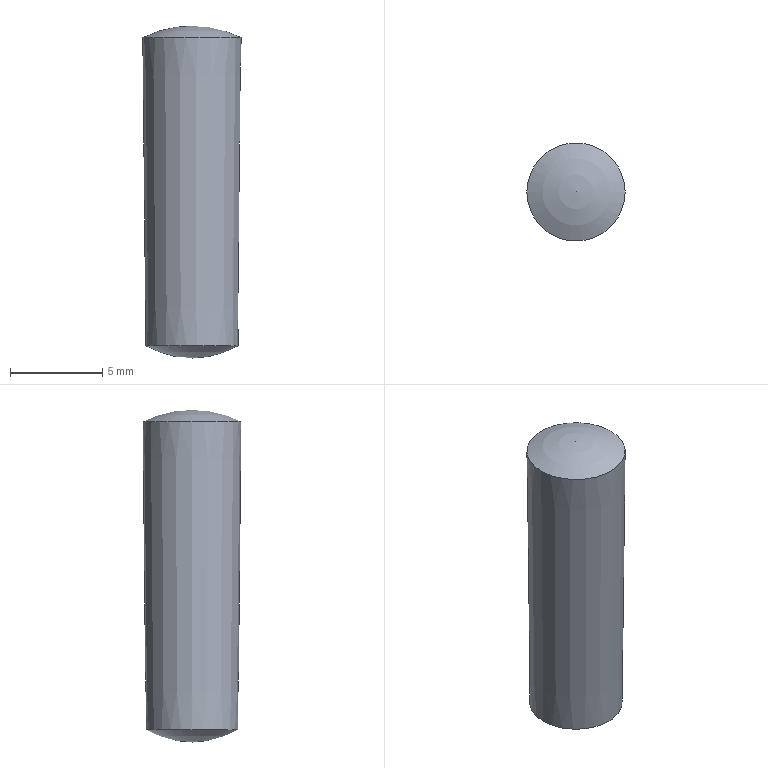Component | NX | GB-T117_A-2000_5X18 | 1 solid | 3 faces | box 5.33 x 5.33 x 18 mm | volume 364 mm3 | sphere 2 | cone 1
STEP:
#1=CARTESIAN_POINT('',(0.,0.,0.));
#2=DIRECTION('',(0.,0.,1.));
#3=DIRECTION('',(1.,0.,0.));
#4=AXIS2_PLACEMENT_3D('',#1,#2,#3);
#5=CARTESIAN_POINT('',(31.561,-84.527,-162.349));
#6=VERTEX_POINT('',#5);
#7=CARTESIAN_POINT('',(34.228,-84.527,-162.349));
#8=DIRECTION('',(0.,0.,-1.));
#9=DIRECTION('',(-1.,0.,0.));
#10=AXIS2_PLACEMENT_3D('',#7,#8,#9);
#11=CIRCLE('',#10,2.667);
#12=CARTESIAN_POINT('',(34.228,-84.527,-167.679));
#13=DIRECTION('',(0.,0.,-1.));
#14=DIRECTION('',(-1.,0.,0.));
#15=AXIS2_PLACEMENT_3D('',#12,#13,#14);
#16=SPHERICAL_SURFACE('',#15,5.96);
#17=CARTESIAN_POINT('',(0.,-1.107));
#18=CARTESIAN_POINT('',(0.0952,-1.107));
#19=CARTESIAN_POINT('',(0.2856,-1.107));
#20=CARTESIAN_POINT('',(0.5712,-1.107));
#21=CARTESIAN_POINT('',(0.8568,-1.107));
#22=CARTESIAN_POINT('',(1.142,-1.107));
#23=CARTESIAN_POINT('',(1.428,-1.107));
#24=CARTESIAN_POINT('',(1.714,-1.107));
#25=CARTESIAN_POINT('',(1.999,-1.107));
#26=CARTESIAN_POINT('',(2.285,-1.107));
#27=CARTESIAN_POINT('',(2.57,-1.107));
#28=CARTESIAN_POINT('',(2.856,-1.107));
#29=CARTESIAN_POINT('',(3.142,-1.107));
#30=CARTESIAN_POINT('',(3.427,-1.107));
#31=CARTESIAN_POINT('',(3.713,-1.107));
#32=CARTESIAN_POINT('',(3.998,-1.107));
#33=CARTESIAN_POINT('',(4.284,-1.107));
#34=CARTESIAN_POINT('',(4.57,-1.107));
#35=CARTESIAN_POINT('',(4.855,-1.107));
#36=CARTESIAN_POINT('',(5.141,-1.107));
#37=CARTESIAN_POINT('',(5.426,-1.107));
#38=CARTESIAN_POINT('',(5.712,-1.107));
#39=CARTESIAN_POINT('',(5.998,-1.107));
#40=CARTESIAN_POINT('',(6.188,-1.107));
#41=CARTESIAN_POINT('',(6.283,-1.107));
#42=B_SPLINE_CURVE_WITH_KNOTS('',3,(#17,#18,#19,#20,#21,#22,#23,#24,#25,#26,#27,#28,#29,#30,#31,#32,#33,#34,#35,#36,#37,#38,#39,#40,#41),.UNSPECIFIED.,.F.,.F.,(4,1,1,1,1,1,1,1,1,1,1,1,1,1,1,1,1,1,1,1,1,1,4),(0.,0.2856,0.5712,0.8568,1.142,1.428,1.714,1.999,2.285,2.57,2.856,3.142,3.427,3.713,3.998,4.284,4.57,4.855,5.141,5.426,5.712,5.998,6.283),.QUASI_UNIFORM_KNOTS.);
#43=(GEOMETRIC_REPRESENTATION_CONTEXT(2)PARAMETRIC_REPRESENTATION_CONTEXT()REPRESENTATION_CONTEXT('',''));
#44=DEFINITIONAL_REPRESENTATION('',(#42),#43);
#45=PCURVE('',#16,#44);
#46=CARTESIAN_POINT('',(34.228,-84.527,-162.349));
#47=DIRECTION('',(0.,0.,1.));
#48=DIRECTION('',(1.,0.,0.));
#49=AXIS2_PLACEMENT_3D('',#46,#47,#48);
#50=CONICAL_SURFACE('',#49,2.667,0.01);
#51=CARTESIAN_POINT('',(9.425,0.));
#52=DIRECTION('',(-1.,0.));
#53=VECTOR('',#52,1.);
#54=LINE('',#51,#53);
#55=(GEOMETRIC_REPRESENTATION_CONTEXT(2)PARAMETRIC_REPRESENTATION_CONTEXT()REPRESENTATION_CONTEXT('',''));
#56=DEFINITIONAL_REPRESENTATION('',(#54),#55);
#57=PCURVE('',#50,#56);
#58=SURFACE_CURVE('',#11,(#45,#57),.PCURVE_S1.);
#59=EDGE_CURVE('',#6,#6,#58,.T.);
#60=ORIENTED_EDGE('',*,*,#59,.F.);
#61=CARTESIAN_POINT('',(34.228,-84.527,-161.719));
#62=VERTEX_POINT('',#61);
#63=CARTESIAN_POINT('',(34.228,-84.527,-161.719));
#64=CARTESIAN_POINT('',(33.537,-84.527,-161.719));
#65=CARTESIAN_POINT('',(32.846,-84.527,-161.826));
#66=CARTESIAN_POINT('',(32.179,-84.527,-162.04));
#67=CARTESIAN_POINT('',(31.561,-84.527,-162.349));
#68=B_SPLINE_CURVE_WITH_KNOTS('',4,(#63,#64,#65,#66,#67),.UNSPECIFIED.,.F.,.F.,(5,5),(-1.571,-1.107),.PIECEWISE_BEZIER_KNOTS.);
#69=CARTESIAN_POINT('',(0.,0.));
#70=DIRECTION('',(0.,1.));
#71=VECTOR('',#70,1.);
#72=LINE('',#69,#71);
#73=(GEOMETRIC_REPRESENTATION_CONTEXT(2)PARAMETRIC_REPRESENTATION_CONTEXT()REPRESENTATION_CONTEXT('',''));
#74=DEFINITIONAL_REPRESENTATION('',(#72),#73);
#75=PCURVE('',#16,#74);
#76=CARTESIAN_POINT('',(6.283,0.));
#77=DIRECTION('',(0.,1.));
#78=VECTOR('',#77,1.);
#79=LINE('',#76,#78);
#80=(GEOMETRIC_REPRESENTATION_CONTEXT(2)PARAMETRIC_REPRESENTATION_CONTEXT()REPRESENTATION_CONTEXT('',''));
#81=DEFINITIONAL_REPRESENTATION('',(#79),#80);
#82=PCURVE('',#16,#81);
#83=SEAM_CURVE('',#68,(#75,#82),.PCURVE_S1.);
#84=EDGE_CURVE('',#62,#6,#83,.T.);
#85=ORIENTED_EDGE('',*,*,#84,.F.);
#86=ORIENTED_EDGE('',*,*,#84,.T.);
#87=EDGE_LOOP('',(#60,#85,#86));
#88=FACE_BOUND('',#87,.T.);
#89=ADVANCED_FACE('',(#88),#16,.T.);
#90=CARTESIAN_POINT('',(31.728,-84.527,-179.049));
#91=VERTEX_POINT('',#90);
#92=CARTESIAN_POINT('',(36.728,-84.527,-179.049));
#93=VERTEX_POINT('',#92);
#94=CARTESIAN_POINT('',(34.228,-84.527,-179.049));
#95=DIRECTION('',(0.,0.,-1.));
#96=DIRECTION('',(-1.,0.,0.));
#97=AXIS2_PLACEMENT_3D('',#94,#95,#96);
#98=CIRCLE('',#97,2.5);
#99=CARTESIAN_POINT('',(9.425,-16.7));
#100=DIRECTION('',(-1.,0.));
#101=VECTOR('',#100,1.);
#102=LINE('',#99,#101);
#103=(GEOMETRIC_REPRESENTATION_CONTEXT(2)PARAMETRIC_REPRESENTATION_CONTEXT()REPRESENTATION_CONTEXT('',''));
#104=DEFINITIONAL_REPRESENTATION('',(#102),#103);
#105=PCURVE('',#50,#104);
#106=CARTESIAN_POINT('',(34.228,-84.527,-174.719));
#107=DIRECTION('',(0.,0.,-1.));
#108=DIRECTION('',(1.,0.,0.));
#109=AXIS2_PLACEMENT_3D('',#106,#107,#108);
#110=SPHERICAL_SURFACE('',#109,5.);
#111=CARTESIAN_POINT('',(3.142,1.047));
#112=CARTESIAN_POINT('',(3.237,1.047));
#113=CARTESIAN_POINT('',(3.427,1.047));
#114=CARTESIAN_POINT('',(3.713,1.047));
#115=CARTESIAN_POINT('',(3.998,1.047));
#116=CARTESIAN_POINT('',(4.284,1.047));
#117=CARTESIAN_POINT('',(4.57,1.047));
#118=CARTESIAN_POINT('',(4.855,1.047));
#119=CARTESIAN_POINT('',(5.141,1.047));
#120=CARTESIAN_POINT('',(5.426,1.047));
#121=CARTESIAN_POINT('',(5.712,1.047));
#122=CARTESIAN_POINT('',(5.998,1.047));
#123=CARTESIAN_POINT('',(6.283,1.047));
#124=CARTESIAN_POINT('',(6.569,1.047));
#125=CARTESIAN_POINT('',(6.854,1.047));
#126=CARTESIAN_POINT('',(7.14,1.047));
#127=CARTESIAN_POINT('',(7.426,1.047));
#128=CARTESIAN_POINT('',(7.711,1.047));
#129=CARTESIAN_POINT('',(7.997,1.047));
#130=CARTESIAN_POINT('',(8.282,1.047));
#131=CARTESIAN_POINT('',(8.568,1.047));
#132=CARTESIAN_POINT('',(8.854,1.047));
#133=CARTESIAN_POINT('',(9.139,1.047));
#134=CARTESIAN_POINT('',(9.33,1.047));
#135=CARTESIAN_POINT('',(9.425,1.047));
#136=B_SPLINE_CURVE_WITH_KNOTS('',3,(#111,#112,#113,#114,#115,#116,#117,#118,#119,#120,#121,#122,#123,#124,#125,#126,#127,#128,#129,#130,#131,#132,#133,#134,#135),.UNSPECIFIED.,.F.,.F.,(4,1,1,1,1,1,1,1,1,1,1,1,1,1,1,1,1,1,1,1,1,1,4),(0.,0.2856,0.5712,0.8568,1.142,1.428,1.714,1.999,2.285,2.57,2.856,3.142,3.427,3.713,3.998,4.284,4.57,4.855,5.141,5.426,5.712,5.998,6.283),.QUASI_UNIFORM_KNOTS.);
#137=(GEOMETRIC_REPRESENTATION_CONTEXT(2)PARAMETRIC_REPRESENTATION_CONTEXT()REPRESENTATION_CONTEXT('',''));
#138=DEFINITIONAL_REPRESENTATION('',(#136),#137);
#139=PCURVE('',#110,#138);
#140=SURFACE_CURVE('',#98,(#105,#139),.PCURVE_S1.);
#141=EDGE_CURVE('',#91,#93,#140,.T.);
#142=ORIENTED_EDGE('',*,*,#141,.F.);
#143=CARTESIAN_POINT('',(31.728,-84.527,-179.049));
#144=CARTESIAN_POINT('',(31.561,-84.527,-162.349));
#145=B_SPLINE_CURVE_WITH_KNOTS('',1,(#143,#144),.UNSPECIFIED.,.F.,.F.,(2,2),(-16.701,0.),.PIECEWISE_BEZIER_KNOTS.);
#146=CARTESIAN_POINT('',(9.425,0.));
#147=DIRECTION('',(0.,1.));
#148=VECTOR('',#147,1.);
#149=LINE('',#146,#148);
#150=(GEOMETRIC_REPRESENTATION_CONTEXT(2)PARAMETRIC_REPRESENTATION_CONTEXT()REPRESENTATION_CONTEXT('',''));
#151=DEFINITIONAL_REPRESENTATION('',(#149),#150);
#152=PCURVE('',#50,#151);
#153=CARTESIAN_POINT('',(3.142,0.));
#154=DIRECTION('',(0.,1.));
#155=VECTOR('',#154,1.);
#156=LINE('',#153,#155);
#157=(GEOMETRIC_REPRESENTATION_CONTEXT(2)PARAMETRIC_REPRESENTATION_CONTEXT()REPRESENTATION_CONTEXT('',''));
#158=DEFINITIONAL_REPRESENTATION('',(#156),#157);
#159=PCURVE('',#50,#158);
#160=SEAM_CURVE('',#145,(#152,#159),.PCURVE_S1.);
#161=EDGE_CURVE('',#91,#6,#160,.T.);
#162=ORIENTED_EDGE('',*,*,#161,.T.);
#163=ORIENTED_EDGE('',*,*,#59,.T.);
#164=ORIENTED_EDGE('',*,*,#161,.F.);
#165=CARTESIAN_POINT('',(34.228,-84.527,-179.049));
#166=DIRECTION('',(0.,0.,-1.));
#167=DIRECTION('',(-1.,0.,0.));
#168=AXIS2_PLACEMENT_3D('',#165,#166,#167);
#169=CIRCLE('',#168,2.5);
#170=CARTESIAN_POINT('',(9.425,-16.7));
#171=DIRECTION('',(-1.,0.));
#172=VECTOR('',#171,1.);
#173=LINE('',#170,#172);
#174=(GEOMETRIC_REPRESENTATION_CONTEXT(2)PARAMETRIC_REPRESENTATION_CONTEXT()REPRESENTATION_CONTEXT('',''));
#175=DEFINITIONAL_REPRESENTATION('',(#173),#174);
#176=PCURVE('',#50,#175);
#177=CARTESIAN_POINT('',(-3.142,1.047));
#178=CARTESIAN_POINT('',(-3.046,1.047));
#179=CARTESIAN_POINT('',(-2.856,1.047));
#180=CARTESIAN_POINT('',(-2.57,1.047));
#181=CARTESIAN_POINT('',(-2.285,1.047));
#182=CARTESIAN_POINT('',(-1.999,1.047));
#183=CARTESIAN_POINT('',(-1.714,1.047));
#184=CARTESIAN_POINT('',(-1.428,1.047));
#185=CARTESIAN_POINT('',(-1.142,1.047));
#186=CARTESIAN_POINT('',(-0.8568,1.047));
#187=CARTESIAN_POINT('',(-0.5712,1.047));
#188=CARTESIAN_POINT('',(-0.2856,1.047));
#189=CARTESIAN_POINT('',(0.,1.047));
#190=CARTESIAN_POINT('',(0.2856,1.047));
#191=CARTESIAN_POINT('',(0.5712,1.047));
#192=CARTESIAN_POINT('',(0.8568,1.047));
#193=CARTESIAN_POINT('',(1.142,1.047));
#194=CARTESIAN_POINT('',(1.428,1.047));
#195=CARTESIAN_POINT('',(1.714,1.047));
#196=CARTESIAN_POINT('',(1.999,1.047));
#197=CARTESIAN_POINT('',(2.285,1.047));
#198=CARTESIAN_POINT('',(2.57,1.047));
#199=CARTESIAN_POINT('',(2.856,1.047));
#200=CARTESIAN_POINT('',(3.046,1.047));
#201=CARTESIAN_POINT('',(3.142,1.047));
#202=B_SPLINE_CURVE_WITH_KNOTS('',3,(#177,#178,#179,#180,#181,#182,#183,#184,#185,#186,#187,#188,#189,#190,#191,#192,#193,#194,#195,#196,#197,#198,#199,#200,#201),.UNSPECIFIED.,.F.,.F.,(4,1,1,1,1,1,1,1,1,1,1,1,1,1,1,1,1,1,1,1,1,1,4),(0.,0.2856,0.5712,0.8568,1.142,1.428,1.714,1.999,2.285,2.57,2.856,3.142,3.427,3.713,3.998,4.284,4.57,4.855,5.141,5.426,5.712,5.998,6.283),.QUASI_UNIFORM_KNOTS.);
#203=(GEOMETRIC_REPRESENTATION_CONTEXT(2)PARAMETRIC_REPRESENTATION_CONTEXT()REPRESENTATION_CONTEXT('',''));
#204=DEFINITIONAL_REPRESENTATION('',(#202),#203);
#205=PCURVE('',#110,#204);
#206=SURFACE_CURVE('',#169,(#176,#205),.PCURVE_S1.);
#207=EDGE_CURVE('',#93,#91,#206,.T.);
#208=ORIENTED_EDGE('',*,*,#207,.F.);
#209=EDGE_LOOP('',(#142,#162,#163,#164,#208));
#210=FACE_BOUND('',#209,.T.);
#211=ADVANCED_FACE('',(#210),#50,.T.);
#212=ORIENTED_EDGE('',*,*,#141,.T.);
#213=CARTESIAN_POINT('',(34.228,-84.527,-179.719));
#214=VERTEX_POINT('',#213);
#215=CARTESIAN_POINT('',(36.728,-84.527,-179.049));
#216=CARTESIAN_POINT('',(36.275,-84.527,-179.311));
#217=CARTESIAN_POINT('',(35.787,-84.527,-179.514));
#218=CARTESIAN_POINT('',(35.275,-84.527,-179.651));
#219=CARTESIAN_POINT('',(34.752,-84.527,-179.719));
#220=CARTESIAN_POINT('',(34.228,-84.527,-179.719));
#221=B_SPLINE_CURVE_WITH_KNOTS('',5,(#215,#216,#217,#218,#219,#220),.UNSPECIFIED.,.F.,.F.,(6,6),(1.047,1.571),.PIECEWISE_BEZIER_KNOTS.);
#222=CARTESIAN_POINT('',(6.283,0.));
#223=DIRECTION('',(0.,1.));
#224=VECTOR('',#223,1.);
#225=LINE('',#222,#224);
#226=(GEOMETRIC_REPRESENTATION_CONTEXT(2)PARAMETRIC_REPRESENTATION_CONTEXT()REPRESENTATION_CONTEXT('',''));
#227=DEFINITIONAL_REPRESENTATION('',(#225),#226);
#228=PCURVE('',#110,#227);
#229=CARTESIAN_POINT('',(0.,0.));
#230=DIRECTION('',(0.,1.));
#231=VECTOR('',#230,1.);
#232=LINE('',#229,#231);
#233=(GEOMETRIC_REPRESENTATION_CONTEXT(2)PARAMETRIC_REPRESENTATION_CONTEXT()REPRESENTATION_CONTEXT('',''));
#234=DEFINITIONAL_REPRESENTATION('',(#232),#233);
#235=PCURVE('',#110,#234);
#236=SEAM_CURVE('',#221,(#228,#235),.PCURVE_S1.);
#237=EDGE_CURVE('',#93,#214,#236,.T.);
#238=ORIENTED_EDGE('',*,*,#237,.T.);
#239=ORIENTED_EDGE('',*,*,#237,.F.);
#240=ORIENTED_EDGE('',*,*,#207,.T.);
#241=EDGE_LOOP('',(#212,#238,#239,#240));
#242=FACE_BOUND('',#241,.T.);
#243=ADVANCED_FACE('',(#242),#110,.T.);
#244=CLOSED_SHELL('',(#89,#211,#243));
#245=MANIFOLD_SOLID_BREP('',#244);
#246=(LENGTH_UNIT()NAMED_UNIT(*)SI_UNIT(.MILLI.,.METRE.));
#247=UNCERTAINTY_MEASURE_WITH_UNIT(LENGTH_MEASURE(0.00001),#246,'','');
#248=(NAMED_UNIT(*)PLANE_ANGLE_UNIT()SI_UNIT($,.RADIAN.));
#249=(NAMED_UNIT(*)SI_UNIT($,.STERADIAN.)SOLID_ANGLE_UNIT());
#250=(GEOMETRIC_REPRESENTATION_CONTEXT(3)GLOBAL_UNCERTAINTY_ASSIGNED_CONTEXT((#247))GLOBAL_UNIT_ASSIGNED_CONTEXT((#246,#248,#249))REPRESENTATION_CONTEXT('',''));
#251=ADVANCED_BREP_SHAPE_REPRESENTATION('',(#4,#245),#250);